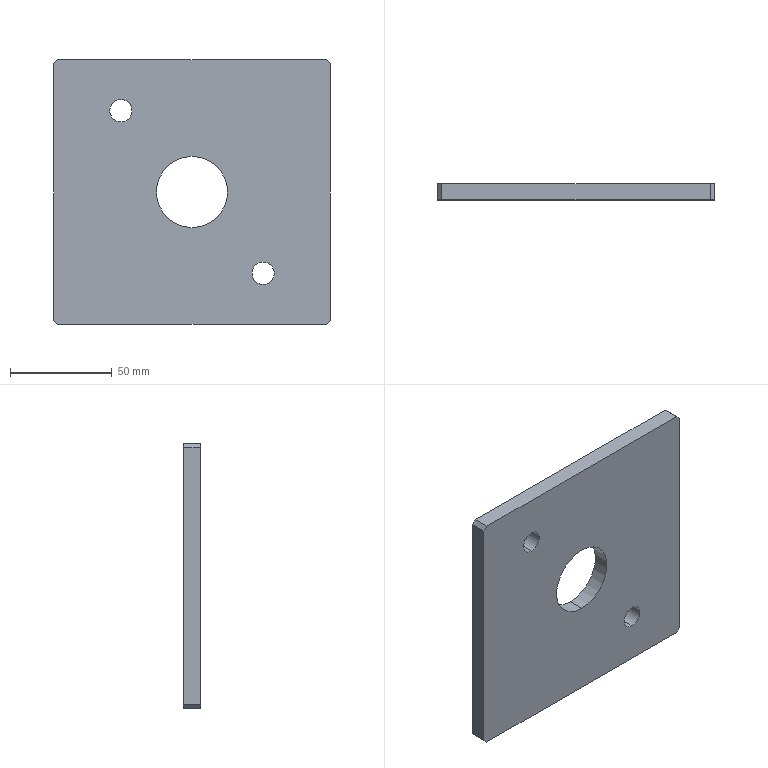Component | SolidWorks | DualStationFixture-1_DualStationFixturePlate-2 | 1 solid | 16 faces | box 136 x 8 x 130 mm | volume 132159 mm3 | plane 10 | cylinder 6 | commonest cylinder face diameters 11 x4 35 x2
build123d program:
from build123d import *

# Parameters (mm, degrees)
SKETCH1_W           = 130
SKETCH1_H           = 136
BOSS_EXTRUDE1_DEPTH = 4
SKETCH2_R           = 17.5
CUT_EXTRUDE1_DEPTH  = 10
CHAMFER1_SIZE       = 2
SKETCH3_R           = 5.5
CUT_EXTRUDE2_DEPTH  = 95.409


with BuildPart() as part:
    # Sketch1 → Boss-Extrude1 (new, symmetric)
    with BuildSketch(Plane.XY):
        Rectangle(SKETCH1_W, SKETCH1_H)
    extrude(amount=BOSS_EXTRUDE1_DEPTH, both=True)

    # Sketch2 → Cut-Extrude1 (cut)
    with BuildSketch(Plane.XY.offset(4)):
        Circle(SKETCH2_R)
    extrude(amount=-CUT_EXTRUDE1_DEPTH, mode=Mode.SUBTRACT)

    # Chamfer1
    chamfer1_edges = [part.edges().sort_by_distance(p)[0] for p in [
        (-65, 68, 0),
        (65, 68, 0),
        (65, -68, 0),
        (-65, -68, 0),
    ]]
    chamfer(chamfer1_edges, length=CHAMFER1_SIZE)

    # Sketch3 → Cut-Extrude2 (cut, through all)
    with BuildSketch(Plane.XY.offset(4)):
        with Locations((-40, 35)):
            Circle(SKETCH3_R)
        with Locations((40, -35)):
            Circle(SKETCH3_R)
    extrude(amount=-CUT_EXTRUDE2_DEPTH, mode=Mode.SUBTRACT)


solid = part.part

# Placed as in the assembly
solid = solid.moved(Location((191.898, 373.813, 99.048), (-90, 0, 90)))
STEP:
#1=COLOUR_RGB('',0.7922,0.8196,0.9333);
#2=FILL_AREA_STYLE_COLOUR('',#1);
#3=FILL_AREA_STYLE('',(#2));
#4=SURFACE_STYLE_FILL_AREA(#3);
#5=SURFACE_SIDE_STYLE('',(#4));
#6=SURFACE_STYLE_USAGE(.BOTH.,#5);
#7=PRESENTATION_STYLE_ASSIGNMENT((#6));
#8=CARTESIAN_POINT('',(8.933,14.56,2.541));
#9=VERTEX_POINT('',#8);
#10=CARTESIAN_POINT('',(8.933,14.56,2.108));
#11=VERTEX_POINT('',#10);
#12=CARTESIAN_POINT('',(8.933,14.56,2.325));
#13=DIRECTION('',(0.,1.,-0.));
#14=DIRECTION('',(0.,0.,-1.));
#15=AXIS2_PLACEMENT_3D('',#12,#13,#14);
#16=CIRCLE('',#15,0.2165);
#17=EDGE_CURVE('',#9,#11,#16,.T.);
#18=ORIENTED_EDGE('',*,*,#17,.F.);
#19=CARTESIAN_POINT('',(8.933,14.875,2.541));
#20=VERTEX_POINT('',#19);
#21=CARTESIAN_POINT('',(8.933,14.56,2.541));
#22=DIRECTION('',(0.,1.,-0.));
#23=VECTOR('',#22,39.37);
#24=LINE('',#21,#23);
#25=EDGE_CURVE('',#9,#20,#24,.T.);
#26=ORIENTED_EDGE('',*,*,#25,.T.);
#27=CARTESIAN_POINT('',(8.933,14.875,2.108));
#28=VERTEX_POINT('',#27);
#29=CARTESIAN_POINT('',(8.933,14.875,2.325));
#30=DIRECTION('',(0.,1.,-0.));
#31=DIRECTION('',(0.,0.,-1.));
#32=AXIS2_PLACEMENT_3D('',#29,#30,#31);
#33=CIRCLE('',#32,0.2165);
#34=EDGE_CURVE('',#20,#28,#33,.T.);
#35=ORIENTED_EDGE('',*,*,#34,.T.);
#36=CARTESIAN_POINT('',(8.933,14.56,2.108));
#37=DIRECTION('',(0.,1.,-0.));
#38=VECTOR('',#37,39.37);
#39=LINE('',#36,#38);
#40=EDGE_CURVE('',#11,#28,#39,.T.);
#41=ORIENTED_EDGE('',*,*,#40,.F.);
#42=EDGE_LOOP('',(#18,#26,#35,#41));
#43=FACE_OUTER_BOUND('',#42,.T.);
#44=CARTESIAN_POINT('',(8.933,14.56,2.325));
#45=DIRECTION('',(0.,1.,-0.));
#46=DIRECTION('',(0.,0.,-1.));
#47=AXIS2_PLACEMENT_3D('',#44,#45,#46);
#48=CYLINDRICAL_SURFACE('',#47,0.2165);
#49=ADVANCED_FACE('',(#43),#48,.F.);
#50=CARTESIAN_POINT('',(6.177,14.56,5.691));
#51=VERTEX_POINT('',#50);
#52=CARTESIAN_POINT('',(6.177,14.56,5.258));
#53=VERTEX_POINT('',#52);
#54=CARTESIAN_POINT('',(6.177,14.56,5.474));
#55=DIRECTION('',(0.,1.,-0.));
#56=DIRECTION('',(0.,0.,-1.));
#57=AXIS2_PLACEMENT_3D('',#54,#55,#56);
#58=CIRCLE('',#57,0.2165);
#59=EDGE_CURVE('',#51,#53,#58,.T.);
#60=ORIENTED_EDGE('',*,*,#59,.F.);
#61=CARTESIAN_POINT('',(6.177,14.875,5.691));
#62=VERTEX_POINT('',#61);
#63=CARTESIAN_POINT('',(6.177,14.56,5.691));
#64=DIRECTION('',(0.,1.,-0.));
#65=VECTOR('',#64,39.37);
#66=LINE('',#63,#65);
#67=EDGE_CURVE('',#51,#62,#66,.T.);
#68=ORIENTED_EDGE('',*,*,#67,.T.);
#69=CARTESIAN_POINT('',(6.177,14.875,5.258));
#70=VERTEX_POINT('',#69);
#71=CARTESIAN_POINT('',(6.177,14.875,5.474));
#72=DIRECTION('',(0.,1.,-0.));
#73=DIRECTION('',(0.,0.,-1.));
#74=AXIS2_PLACEMENT_3D('',#71,#72,#73);
#75=CIRCLE('',#74,0.2165);
#76=EDGE_CURVE('',#62,#70,#75,.T.);
#77=ORIENTED_EDGE('',*,*,#76,.T.);
#78=CARTESIAN_POINT('',(6.177,14.56,5.258));
#79=DIRECTION('',(0.,1.,-0.));
#80=VECTOR('',#79,39.37);
#81=LINE('',#78,#80);
#82=EDGE_CURVE('',#53,#70,#81,.T.);
#83=ORIENTED_EDGE('',*,*,#82,.F.);
#84=EDGE_LOOP('',(#60,#68,#77,#83));
#85=FACE_OUTER_BOUND('',#84,.T.);
#86=CARTESIAN_POINT('',(6.177,14.56,5.474));
#87=DIRECTION('',(0.,1.,-0.));
#88=DIRECTION('',(0.,0.,-1.));
#89=AXIS2_PLACEMENT_3D('',#86,#87,#88);
#90=CYLINDRICAL_SURFACE('',#89,0.2165);
#91=ADVANCED_FACE('',(#85),#90,.F.);
#92=CARTESIAN_POINT('',(7.555,14.56,4.588));
#93=VERTEX_POINT('',#92);
#94=CARTESIAN_POINT('',(7.555,14.56,3.211));
#95=VERTEX_POINT('',#94);
#96=CARTESIAN_POINT('',(7.555,14.56,3.9));
#97=DIRECTION('',(0.,1.,-0.));
#98=DIRECTION('',(0.,0.,-1.));
#99=AXIS2_PLACEMENT_3D('',#96,#97,#98);
#100=CIRCLE('',#99,0.689);
#101=EDGE_CURVE('',#93,#95,#100,.T.);
#102=ORIENTED_EDGE('',*,*,#101,.F.);
#103=CARTESIAN_POINT('',(7.555,14.875,4.588));
#104=VERTEX_POINT('',#103);
#105=CARTESIAN_POINT('',(7.555,14.481,4.588));
#106=DIRECTION('',(0.,1.,-0.));
#107=VECTOR('',#106,39.37);
#108=LINE('',#105,#107);
#109=EDGE_CURVE('',#93,#104,#108,.T.);
#110=ORIENTED_EDGE('',*,*,#109,.T.);
#111=CARTESIAN_POINT('',(7.555,14.875,3.211));
#112=VERTEX_POINT('',#111);
#113=CARTESIAN_POINT('',(7.555,14.875,3.9));
#114=DIRECTION('',(0.,1.,-0.));
#115=DIRECTION('',(0.,0.,-1.));
#116=AXIS2_PLACEMENT_3D('',#113,#114,#115);
#117=CIRCLE('',#116,0.689);
#118=EDGE_CURVE('',#104,#112,#117,.T.);
#119=ORIENTED_EDGE('',*,*,#118,.T.);
#120=CARTESIAN_POINT('',(7.555,14.481,3.211));
#121=DIRECTION('',(0.,1.,-0.));
#122=VECTOR('',#121,39.37);
#123=LINE('',#120,#122);
#124=EDGE_CURVE('',#95,#112,#123,.T.);
#125=ORIENTED_EDGE('',*,*,#124,.F.);
#126=EDGE_LOOP('',(#102,#110,#119,#125));
#127=FACE_OUTER_BOUND('',#126,.T.);
#128=CARTESIAN_POINT('',(7.555,14.481,3.9));
#129=DIRECTION('',(0.,1.,-0.));
#130=DIRECTION('',(0.,0.,-1.));
#131=AXIS2_PLACEMENT_3D('',#128,#129,#130);
#132=CYLINDRICAL_SURFACE('',#131,0.689);
#133=ADVANCED_FACE('',(#127),#132,.F.);
#134=CARTESIAN_POINT('',(4.957,14.56,6.459));
#135=VERTEX_POINT('',#134);
#136=CARTESIAN_POINT('',(10.153,14.56,6.459));
#137=VERTEX_POINT('',#136);
#138=CARTESIAN_POINT('',(10.232,14.56,6.459));
#139=DIRECTION('',(1.,-0.,0.));
#140=VECTOR('',#139,39.37);
#141=LINE('',#138,#140);
#142=EDGE_CURVE('',#135,#137,#141,.T.);
#143=ORIENTED_EDGE('',*,*,#142,.T.);
#144=CARTESIAN_POINT('',(10.153,14.875,6.459));
#145=VERTEX_POINT('',#144);
#146=CARTESIAN_POINT('',(10.153,14.875,6.459));
#147=DIRECTION('',(0.,1.,-0.));
#148=VECTOR('',#147,39.37);
#149=LINE('',#146,#148);
#150=EDGE_CURVE('',#137,#145,#149,.T.);
#151=ORIENTED_EDGE('',*,*,#150,.T.);
#152=CARTESIAN_POINT('',(4.957,14.875,6.459));
#153=VERTEX_POINT('',#152);
#154=CARTESIAN_POINT('',(10.232,14.875,6.459));
#155=DIRECTION('',(1.,-0.,0.));
#156=VECTOR('',#155,39.37);
#157=LINE('',#154,#156);
#158=EDGE_CURVE('',#153,#145,#157,.T.);
#159=ORIENTED_EDGE('',*,*,#158,.F.);
#160=CARTESIAN_POINT('',(4.957,14.875,6.459));
#161=DIRECTION('',(-0.,-1.,0.));
#162=VECTOR('',#161,39.37);
#163=LINE('',#160,#162);
#164=EDGE_CURVE('',#153,#135,#163,.T.);
#165=ORIENTED_EDGE('',*,*,#164,.T.);
#166=EDGE_LOOP('',(#143,#151,#159,#165));
#167=FACE_OUTER_BOUND('',#166,.T.);
#168=CARTESIAN_POINT('',(10.232,14.875,6.459));
#169=DIRECTION('',(0.,-0.,-1.));
#170=DIRECTION('',(-0.,-1.,0.));
#171=AXIS2_PLACEMENT_3D('',#168,#169,#170);
#172=PLANE('',#171);
#173=ADVANCED_FACE('',(#167),#172,.F.);
#174=CARTESIAN_POINT('',(10.232,14.56,6.38));
#175=VERTEX_POINT('',#174);
#176=CARTESIAN_POINT('',(10.232,14.56,1.419));
#177=VERTEX_POINT('',#176);
#178=CARTESIAN_POINT('',(10.232,14.56,1.34));
#179=DIRECTION('',(-0.,-0.,-1.));
#180=VECTOR('',#179,39.37);
#181=LINE('',#178,#180);
#182=EDGE_CURVE('',#175,#177,#181,.T.);
#183=ORIENTED_EDGE('',*,*,#182,.T.);
#184=CARTESIAN_POINT('',(10.232,14.875,1.419));
#185=VERTEX_POINT('',#184);
#186=CARTESIAN_POINT('',(10.232,14.875,1.419));
#187=DIRECTION('',(0.,1.,-0.));
#188=VECTOR('',#187,39.37);
#189=LINE('',#186,#188);
#190=EDGE_CURVE('',#177,#185,#189,.T.);
#191=ORIENTED_EDGE('',*,*,#190,.T.);
#192=CARTESIAN_POINT('',(10.232,14.875,6.38));
#193=VERTEX_POINT('',#192);
#194=CARTESIAN_POINT('',(10.232,14.875,1.34));
#195=DIRECTION('',(-0.,-0.,-1.));
#196=VECTOR('',#195,39.37);
#197=LINE('',#194,#196);
#198=EDGE_CURVE('',#193,#185,#197,.T.);
#199=ORIENTED_EDGE('',*,*,#198,.F.);
#200=CARTESIAN_POINT('',(10.232,14.875,6.38));
#201=DIRECTION('',(-0.,-1.,0.));
#202=VECTOR('',#201,39.37);
#203=LINE('',#200,#202);
#204=EDGE_CURVE('',#193,#175,#203,.T.);
#205=ORIENTED_EDGE('',*,*,#204,.T.);
#206=EDGE_LOOP('',(#183,#191,#199,#205));
#207=FACE_OUTER_BOUND('',#206,.T.);
#208=CARTESIAN_POINT('',(10.232,14.875,1.34));
#209=DIRECTION('',(-1.,0.,0.));
#210=DIRECTION('',(0.,0.,1.));
#211=AXIS2_PLACEMENT_3D('',#208,#209,#210);
#212=PLANE('',#211);
#213=ADVANCED_FACE('',(#207),#212,.F.);
#214=CARTESIAN_POINT('',(10.153,14.56,1.34));
#215=VERTEX_POINT('',#214);
#216=CARTESIAN_POINT('',(4.957,14.56,1.34));
#217=VERTEX_POINT('',#216);
#218=CARTESIAN_POINT('',(10.232,14.56,1.34));
#219=DIRECTION('',(-1.,0.,-0.));
#220=VECTOR('',#219,39.37);
#221=LINE('',#218,#220);
#222=EDGE_CURVE('',#215,#217,#221,.T.);
#223=ORIENTED_EDGE('',*,*,#222,.T.);
#224=CARTESIAN_POINT('',(4.957,14.875,1.34));
#225=VERTEX_POINT('',#224);
#226=CARTESIAN_POINT('',(4.957,14.875,1.34));
#227=DIRECTION('',(0.,1.,-0.));
#228=VECTOR('',#227,39.37);
#229=LINE('',#226,#228);
#230=EDGE_CURVE('',#217,#225,#229,.T.);
#231=ORIENTED_EDGE('',*,*,#230,.T.);
#232=CARTESIAN_POINT('',(10.153,14.875,1.34));
#233=VERTEX_POINT('',#232);
#234=CARTESIAN_POINT('',(10.232,14.875,1.34));
#235=DIRECTION('',(-1.,0.,-0.));
#236=VECTOR('',#235,39.37);
#237=LINE('',#234,#236);
#238=EDGE_CURVE('',#233,#225,#237,.T.);
#239=ORIENTED_EDGE('',*,*,#238,.F.);
#240=CARTESIAN_POINT('',(10.153,14.875,1.34));
#241=DIRECTION('',(-0.,-1.,0.));
#242=VECTOR('',#241,39.37);
#243=LINE('',#240,#242);
#244=EDGE_CURVE('',#233,#215,#243,.T.);
#245=ORIENTED_EDGE('',*,*,#244,.T.);
#246=EDGE_LOOP('',(#223,#231,#239,#245));
#247=FACE_OUTER_BOUND('',#246,.T.);
#248=CARTESIAN_POINT('',(10.232,14.875,1.34));
#249=DIRECTION('',(-0.,0.,1.));
#250=DIRECTION('',(0.,1.,-0.));
#251=AXIS2_PLACEMENT_3D('',#248,#249,#250);
#252=PLANE('',#251);
#253=ADVANCED_FACE('',(#247),#252,.F.);
#254=CARTESIAN_POINT('',(4.878,14.875,1.419));
#255=VERTEX_POINT('',#254);
#256=CARTESIAN_POINT('',(4.878,14.875,6.38));
#257=VERTEX_POINT('',#256);
#258=CARTESIAN_POINT('',(4.878,14.875,1.34));
#259=DIRECTION('',(0.,0.,1.));
#260=VECTOR('',#259,39.37);
#261=LINE('',#258,#260);
#262=EDGE_CURVE('',#255,#257,#261,.T.);
#263=ORIENTED_EDGE('',*,*,#262,.F.);
#264=CARTESIAN_POINT('',(4.878,14.56,1.419));
#265=VERTEX_POINT('',#264);
#266=CARTESIAN_POINT('',(4.878,14.875,1.419));
#267=DIRECTION('',(-0.,-1.,0.));
#268=VECTOR('',#267,39.37);
#269=LINE('',#266,#268);
#270=EDGE_CURVE('',#255,#265,#269,.T.);
#271=ORIENTED_EDGE('',*,*,#270,.T.);
#272=CARTESIAN_POINT('',(4.878,14.56,6.38));
#273=VERTEX_POINT('',#272);
#274=CARTESIAN_POINT('',(4.878,14.56,1.34));
#275=DIRECTION('',(0.,0.,1.));
#276=VECTOR('',#275,39.37);
#277=LINE('',#274,#276);
#278=EDGE_CURVE('',#265,#273,#277,.T.);
#279=ORIENTED_EDGE('',*,*,#278,.T.);
#280=CARTESIAN_POINT('',(4.878,14.875,6.38));
#281=DIRECTION('',(0.,1.,-0.));
#282=VECTOR('',#281,39.37);
#283=LINE('',#280,#282);
#284=EDGE_CURVE('',#273,#257,#283,.T.);
#285=ORIENTED_EDGE('',*,*,#284,.T.);
#286=EDGE_LOOP('',(#263,#271,#279,#285));
#287=FACE_OUTER_BOUND('',#286,.T.);
#288=CARTESIAN_POINT('',(4.878,14.875,1.34));
#289=DIRECTION('',(1.,-0.,-0.));
#290=DIRECTION('',(-0.,-0.,-1.));
#291=AXIS2_PLACEMENT_3D('',#288,#289,#290);
#292=PLANE('',#291);
#293=ADVANCED_FACE('',(#287),#292,.F.);
#294=CARTESIAN_POINT('',(8.933,14.875,2.325));
#295=DIRECTION('',(0.,1.,-0.));
#296=DIRECTION('',(0.,0.,-1.));
#297=AXIS2_PLACEMENT_3D('',#294,#295,#296);
#298=CIRCLE('',#297,0.2165);
#299=EDGE_CURVE('',#28,#20,#298,.T.);
#300=ORIENTED_EDGE('',*,*,#299,.F.);
#301=ORIENTED_EDGE('',*,*,#34,.F.);
#302=EDGE_LOOP('',(#300,#301));
#303=FACE_BOUND('',#302,.T.);
#304=CARTESIAN_POINT('',(6.177,14.875,5.474));
#305=DIRECTION('',(0.,1.,-0.));
#306=DIRECTION('',(0.,0.,-1.));
#307=AXIS2_PLACEMENT_3D('',#304,#305,#306);
#308=CIRCLE('',#307,0.2165);
#309=EDGE_CURVE('',#70,#62,#308,.T.);
#310=ORIENTED_EDGE('',*,*,#309,.F.);
#311=ORIENTED_EDGE('',*,*,#76,.F.);
#312=EDGE_LOOP('',(#310,#311));
#313=FACE_BOUND('',#312,.T.);
#314=CARTESIAN_POINT('',(7.555,14.875,3.9));
#315=DIRECTION('',(0.,1.,-0.));
#316=DIRECTION('',(0.,0.,-1.));
#317=AXIS2_PLACEMENT_3D('',#314,#315,#316);
#318=CIRCLE('',#317,0.689);
#319=EDGE_CURVE('',#112,#104,#318,.T.);
#320=ORIENTED_EDGE('',*,*,#319,.F.);
#321=ORIENTED_EDGE('',*,*,#118,.F.);
#322=EDGE_LOOP('',(#320,#321));
#323=FACE_BOUND('',#322,.T.);
#324=ORIENTED_EDGE('',*,*,#238,.T.);
#325=CARTESIAN_POINT('',(4.976,14.875,1.321));
#326=DIRECTION('',(-0.7071,0.,0.7071));
#327=VECTOR('',#326,39.37);
#328=LINE('',#325,#327);
#329=EDGE_CURVE('',#225,#255,#328,.T.);
#330=ORIENTED_EDGE('',*,*,#329,.T.);
#331=ORIENTED_EDGE('',*,*,#262,.T.);
#332=CARTESIAN_POINT('',(4.976,14.875,6.478));
#333=DIRECTION('',(0.7071,-0.,0.7071));
#334=VECTOR('',#333,39.37);
#335=LINE('',#332,#334);
#336=EDGE_CURVE('',#257,#153,#335,.T.);
#337=ORIENTED_EDGE('',*,*,#336,.T.);
#338=ORIENTED_EDGE('',*,*,#158,.T.);
#339=CARTESIAN_POINT('',(10.134,14.875,6.478));
#340=DIRECTION('',(0.7071,-0.,-0.7071));
#341=VECTOR('',#340,39.37);
#342=LINE('',#339,#341);
#343=EDGE_CURVE('',#145,#193,#342,.T.);
#344=ORIENTED_EDGE('',*,*,#343,.T.);
#345=ORIENTED_EDGE('',*,*,#198,.T.);
#346=CARTESIAN_POINT('',(10.134,14.875,1.321));
#347=DIRECTION('',(-0.7071,0.,-0.7071));
#348=VECTOR('',#347,39.37);
#349=LINE('',#346,#348);
#350=EDGE_CURVE('',#185,#233,#349,.T.);
#351=ORIENTED_EDGE('',*,*,#350,.T.);
#352=EDGE_LOOP('',(#324,#330,#331,#337,#338,#344,#345,#351));
#353=FACE_OUTER_BOUND('',#352,.T.);
#354=CARTESIAN_POINT('',(7.555,14.875,3.9));
#355=DIRECTION('',(0.,1.,-0.));
#356=DIRECTION('',(0.,-0.,-1.));
#357=AXIS2_PLACEMENT_3D('',#354,#355,#356);
#358=PLANE('',#357);
#359=ADVANCED_FACE('',(#303,#313,#323,#353),#358,.T.);
#360=CARTESIAN_POINT('',(8.933,14.56,2.325));
#361=DIRECTION('',(0.,1.,-0.));
#362=DIRECTION('',(0.,0.,-1.));
#363=AXIS2_PLACEMENT_3D('',#360,#361,#362);
#364=CIRCLE('',#363,0.2165);
#365=EDGE_CURVE('',#11,#9,#364,.T.);
#366=ORIENTED_EDGE('',*,*,#365,.T.);
#367=ORIENTED_EDGE('',*,*,#17,.T.);
#368=EDGE_LOOP('',(#366,#367));
#369=FACE_BOUND('',#368,.T.);
#370=CARTESIAN_POINT('',(6.177,14.56,5.474));
#371=DIRECTION('',(0.,1.,-0.));
#372=DIRECTION('',(0.,0.,-1.));
#373=AXIS2_PLACEMENT_3D('',#370,#371,#372);
#374=CIRCLE('',#373,0.2165);
#375=EDGE_CURVE('',#53,#51,#374,.T.);
#376=ORIENTED_EDGE('',*,*,#375,.T.);
#377=ORIENTED_EDGE('',*,*,#59,.T.);
#378=EDGE_LOOP('',(#376,#377));
#379=FACE_BOUND('',#378,.T.);
#380=CARTESIAN_POINT('',(7.555,14.56,3.9));
#381=DIRECTION('',(0.,1.,-0.));
#382=DIRECTION('',(0.,0.,-1.));
#383=AXIS2_PLACEMENT_3D('',#380,#381,#382);
#384=CIRCLE('',#383,0.689);
#385=EDGE_CURVE('',#95,#93,#384,.T.);
#386=ORIENTED_EDGE('',*,*,#385,.T.);
#387=ORIENTED_EDGE('',*,*,#101,.T.);
#388=EDGE_LOOP('',(#386,#387));
#389=FACE_BOUND('',#388,.T.);
#390=ORIENTED_EDGE('',*,*,#278,.F.);
#391=CARTESIAN_POINT('',(4.878,14.56,1.419));
#392=DIRECTION('',(0.7071,-0.,-0.7071));
#393=VECTOR('',#392,39.37);
#394=LINE('',#391,#393);
#395=EDGE_CURVE('',#265,#217,#394,.T.);
#396=ORIENTED_EDGE('',*,*,#395,.T.);
#397=ORIENTED_EDGE('',*,*,#222,.F.);
#398=CARTESIAN_POINT('',(10.153,14.56,1.34));
#399=DIRECTION('',(0.7071,-0.,0.7071));
#400=VECTOR('',#399,39.37);
#401=LINE('',#398,#400);
#402=EDGE_CURVE('',#215,#177,#401,.T.);
#403=ORIENTED_EDGE('',*,*,#402,.T.);
#404=ORIENTED_EDGE('',*,*,#182,.F.);
#405=CARTESIAN_POINT('',(10.232,14.56,6.38));
#406=DIRECTION('',(-0.7071,0.,0.7071));
#407=VECTOR('',#406,39.37);
#408=LINE('',#405,#407);
#409=EDGE_CURVE('',#175,#137,#408,.T.);
#410=ORIENTED_EDGE('',*,*,#409,.T.);
#411=ORIENTED_EDGE('',*,*,#142,.F.);
#412=CARTESIAN_POINT('',(4.957,14.56,6.459));
#413=DIRECTION('',(-0.7071,0.,-0.7071));
#414=VECTOR('',#413,39.37);
#415=LINE('',#412,#414);
#416=EDGE_CURVE('',#135,#273,#415,.T.);
#417=ORIENTED_EDGE('',*,*,#416,.T.);
#418=EDGE_LOOP('',(#390,#396,#397,#403,#404,#410,#411,#417));
#419=FACE_OUTER_BOUND('',#418,.T.);
#420=CARTESIAN_POINT('',(7.555,14.56,3.9));
#421=DIRECTION('',(0.,1.,-0.));
#422=DIRECTION('',(0.,-0.,-1.));
#423=AXIS2_PLACEMENT_3D('',#420,#421,#422);
#424=PLANE('',#423);
#425=ADVANCED_FACE('',(#369,#379,#389,#419),#424,.F.);
#426=ORIENTED_EDGE('',*,*,#109,.F.);
#427=ORIENTED_EDGE('',*,*,#385,.F.);
#428=ORIENTED_EDGE('',*,*,#124,.T.);
#429=ORIENTED_EDGE('',*,*,#319,.T.);
#430=EDGE_LOOP('',(#426,#427,#428,#429));
#431=FACE_OUTER_BOUND('',#430,.T.);
#432=CARTESIAN_POINT('',(7.555,14.481,3.9));
#433=DIRECTION('',(0.,1.,-0.));
#434=DIRECTION('',(0.,0.,-1.));
#435=AXIS2_PLACEMENT_3D('',#432,#433,#434);
#436=CYLINDRICAL_SURFACE('',#435,0.689);
#437=ADVANCED_FACE('',(#431),#436,.F.);
#438=ORIENTED_EDGE('',*,*,#329,.F.);
#439=ORIENTED_EDGE('',*,*,#230,.F.);
#440=ORIENTED_EDGE('',*,*,#395,.F.);
#441=ORIENTED_EDGE('',*,*,#270,.F.);
#442=EDGE_LOOP('',(#438,#439,#440,#441));
#443=FACE_OUTER_BOUND('',#442,.T.);
#444=CARTESIAN_POINT('',(4.878,14.875,1.419));
#445=DIRECTION('',(0.7071,-0.,0.7071));
#446=DIRECTION('',(-0.,-1.,0.));
#447=AXIS2_PLACEMENT_3D('',#444,#445,#446);
#448=PLANE('',#447);
#449=ADVANCED_FACE('',(#443),#448,.F.);
#450=ORIENTED_EDGE('',*,*,#350,.F.);
#451=ORIENTED_EDGE('',*,*,#190,.F.);
#452=ORIENTED_EDGE('',*,*,#402,.F.);
#453=ORIENTED_EDGE('',*,*,#244,.F.);
#454=EDGE_LOOP('',(#450,#451,#452,#453));
#455=FACE_OUTER_BOUND('',#454,.T.);
#456=CARTESIAN_POINT('',(10.153,14.875,1.34));
#457=DIRECTION('',(-0.7071,0.,0.7071));
#458=DIRECTION('',(-0.,-1.,0.));
#459=AXIS2_PLACEMENT_3D('',#456,#457,#458);
#460=PLANE('',#459);
#461=ADVANCED_FACE('',(#455),#460,.F.);
#462=ORIENTED_EDGE('',*,*,#343,.F.);
#463=ORIENTED_EDGE('',*,*,#150,.F.);
#464=ORIENTED_EDGE('',*,*,#409,.F.);
#465=ORIENTED_EDGE('',*,*,#204,.F.);
#466=EDGE_LOOP('',(#462,#463,#464,#465));
#467=FACE_OUTER_BOUND('',#466,.T.);
#468=CARTESIAN_POINT('',(10.232,14.875,6.38));
#469=DIRECTION('',(-0.7071,0.,-0.7071));
#470=DIRECTION('',(-0.,-1.,0.));
#471=AXIS2_PLACEMENT_3D('',#468,#469,#470);
#472=PLANE('',#471);
#473=ADVANCED_FACE('',(#467),#472,.F.);
#474=ORIENTED_EDGE('',*,*,#336,.F.);
#475=ORIENTED_EDGE('',*,*,#284,.F.);
#476=ORIENTED_EDGE('',*,*,#416,.F.);
#477=ORIENTED_EDGE('',*,*,#164,.F.);
#478=EDGE_LOOP('',(#474,#475,#476,#477));
#479=FACE_OUTER_BOUND('',#478,.T.);
#480=CARTESIAN_POINT('',(4.957,14.875,6.459));
#481=DIRECTION('',(0.7071,-0.,-0.7071));
#482=DIRECTION('',(-0.,-1.,0.));
#483=AXIS2_PLACEMENT_3D('',#480,#481,#482);
#484=PLANE('',#483);
#485=ADVANCED_FACE('',(#479),#484,.F.);
#486=ORIENTED_EDGE('',*,*,#67,.F.);
#487=ORIENTED_EDGE('',*,*,#375,.F.);
#488=ORIENTED_EDGE('',*,*,#82,.T.);
#489=ORIENTED_EDGE('',*,*,#309,.T.);
#490=EDGE_LOOP('',(#486,#487,#488,#489));
#491=FACE_OUTER_BOUND('',#490,.T.);
#492=CARTESIAN_POINT('',(6.177,14.56,5.474));
#493=DIRECTION('',(0.,1.,-0.));
#494=DIRECTION('',(0.,0.,-1.));
#495=AXIS2_PLACEMENT_3D('',#492,#493,#494);
#496=CYLINDRICAL_SURFACE('',#495,0.2165);
#497=ADVANCED_FACE('',(#491),#496,.F.);
#498=ORIENTED_EDGE('',*,*,#25,.F.);
#499=ORIENTED_EDGE('',*,*,#365,.F.);
#500=ORIENTED_EDGE('',*,*,#40,.T.);
#501=ORIENTED_EDGE('',*,*,#299,.T.);
#502=EDGE_LOOP('',(#498,#499,#500,#501));
#503=FACE_OUTER_BOUND('',#502,.T.);
#504=CARTESIAN_POINT('',(8.933,14.56,2.325));
#505=DIRECTION('',(0.,1.,-0.));
#506=DIRECTION('',(0.,0.,-1.));
#507=AXIS2_PLACEMENT_3D('',#504,#505,#506);
#508=CYLINDRICAL_SURFACE('',#507,0.2165);
#509=ADVANCED_FACE('',(#503),#508,.F.);
#510=CLOSED_SHELL('',(#49,#91,#133,#173,#213,#253,#293,#359,#425,#437,#449,#461,#473,#485,#497,#509));
#511=MANIFOLD_SOLID_BREP('',#510);
#512=STYLED_ITEM('',(#7),#511);
#513=(LENGTH_UNIT()NAMED_UNIT(*)SI_UNIT($,.METRE.));
#514=LENGTH_MEASURE_WITH_UNIT(LENGTH_MEASURE(0.0254),#513);
#515=DIMENSIONAL_EXPONENTS(1.,0.,0.,0.,0.,0.,0.);
#516=(CONVERSION_BASED_UNIT('',#514)LENGTH_UNIT()NAMED_UNIT(#515));
#517=UNCERTAINTY_MEASURE_WITH_UNIT(LENGTH_MEASURE(0.00001),#516,'','');
#518=(NAMED_UNIT(*)PLANE_ANGLE_UNIT()SI_UNIT($,.RADIAN.));
#519=(NAMED_UNIT(*)SI_UNIT($,.STERADIAN.)SOLID_ANGLE_UNIT());
#520=(GEOMETRIC_REPRESENTATION_CONTEXT(3)GLOBAL_UNCERTAINTY_ASSIGNED_CONTEXT((#517))GLOBAL_UNIT_ASSIGNED_CONTEXT((#516,#518,#519))REPRESENTATION_CONTEXT('',''));
#521=MECHANICAL_DESIGN_GEOMETRIC_PRESENTATION_REPRESENTATION('',(#512),#520);
#522=CARTESIAN_POINT('',(0.,0.,0.));
#523=DIRECTION('',(0.,0.,1.));
#524=DIRECTION('',(1.,0.,0.));
#525=AXIS2_PLACEMENT_3D('',#522,#523,#524);
#526=(LENGTH_UNIT()NAMED_UNIT(*)SI_UNIT($,.METRE.));
#527=LENGTH_MEASURE_WITH_UNIT(LENGTH_MEASURE(0.0254),#526);
#528=DIMENSIONAL_EXPONENTS(1.,0.,0.,0.,0.,0.,0.);
#529=(CONVERSION_BASED_UNIT('',#527)LENGTH_UNIT()NAMED_UNIT(#528));
#530=UNCERTAINTY_MEASURE_WITH_UNIT(LENGTH_MEASURE(0.00001),#529,'','');
#531=(NAMED_UNIT(*)PLANE_ANGLE_UNIT()SI_UNIT($,.RADIAN.));
#532=(NAMED_UNIT(*)SI_UNIT($,.STERADIAN.)SOLID_ANGLE_UNIT());
#533=(GEOMETRIC_REPRESENTATION_CONTEXT(3)GLOBAL_UNCERTAINTY_ASSIGNED_CONTEXT((#530))GLOBAL_UNIT_ASSIGNED_CONTEXT((#529,#531,#532))REPRESENTATION_CONTEXT('',''));
#534=ADVANCED_BREP_SHAPE_REPRESENTATION('',(#511,#525),#533);
#535=PRESENTATION_LAYER_ASSIGNMENT('','',(#512));